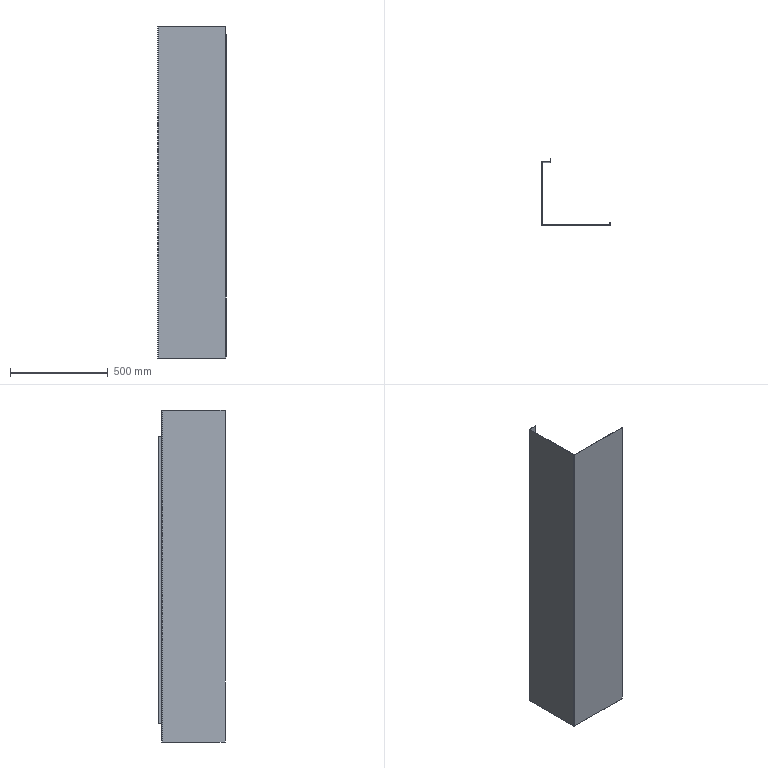Component | SolidWorks | SidePanel-1 | 1 solid | 41 faces | box 350 x 342.5 x 1700 mm | volume 1886748 mm3 | plane 33 | cylinder 8 | commonest cylinder face diameters 1 x4 4 x4
STEP:
#1=COLOUR_RGB('',0.7922,0.8196,0.9333);
#2=FILL_AREA_STYLE_COLOUR('',#1);
#3=FILL_AREA_STYLE('',(#2));
#4=SURFACE_STYLE_FILL_AREA(#3);
#5=SURFACE_SIDE_STYLE('',(#4));
#6=SURFACE_STYLE_USAGE(.BOTH.,#5);
#7=PRESENTATION_STYLE_ASSIGNMENT((#6));
#8=CARTESIAN_POINT('',(7.992,-6.09,65.157));
#9=VERTEX_POINT('',#8);
#10=CARTESIAN_POINT('',(7.992,-6.484,65.157));
#11=VERTEX_POINT('',#10);
#12=CARTESIAN_POINT('',(7.992,-6.563,65.157));
#13=DIRECTION('',(-0.,-1.,0.));
#14=VECTOR('',#13,39.37);
#15=LINE('',#12,#14);
#16=EDGE_CURVE('',#9,#11,#15,.T.);
#17=ORIENTED_EDGE('',*,*,#16,.T.);
#18=CARTESIAN_POINT('',(7.992,-6.484,0.3937));
#19=VERTEX_POINT('',#18);
#20=CARTESIAN_POINT('',(7.992,-6.484,66.929));
#21=DIRECTION('',(0.,0.,-1.));
#22=VECTOR('',#21,39.37);
#23=LINE('',#20,#22);
#24=EDGE_CURVE('',#11,#19,#23,.T.);
#25=ORIENTED_EDGE('',*,*,#24,.T.);
#26=CARTESIAN_POINT('',(7.992,-6.09,0.3937));
#27=VERTEX_POINT('',#26);
#28=CARTESIAN_POINT('',(7.992,-6.563,0.3937));
#29=DIRECTION('',(0.,1.,0.));
#30=VECTOR('',#29,39.37);
#31=LINE('',#28,#30);
#32=EDGE_CURVE('',#19,#27,#31,.T.);
#33=ORIENTED_EDGE('',*,*,#32,.T.);
#34=CARTESIAN_POINT('',(7.992,-6.09,66.929));
#35=DIRECTION('',(0.,0.,-1.));
#36=VECTOR('',#35,39.37);
#37=LINE('',#34,#36);
#38=EDGE_CURVE('',#9,#27,#37,.T.);
#39=ORIENTED_EDGE('',*,*,#38,.F.);
#40=EDGE_LOOP('',(#17,#25,#33,#39));
#41=FACE_OUTER_BOUND('',#40,.T.);
#42=CARTESIAN_POINT('',(7.992,-6.563,66.929));
#43=DIRECTION('',(-1.,0.,0.));
#44=DIRECTION('',(-0.,-1.,0.));
#45=AXIS2_PLACEMENT_3D('',#42,#43,#44);
#46=PLANE('',#45);
#47=ADVANCED_FACE('',(#41),#46,.F.);
#48=CARTESIAN_POINT('',(7.933,-6.09,65.157));
#49=VERTEX_POINT('',#48);
#50=CARTESIAN_POINT('',(7.933,-6.09,0.3937));
#51=VERTEX_POINT('',#50);
#52=CARTESIAN_POINT('',(7.933,-6.09,66.929));
#53=DIRECTION('',(0.,0.,-1.));
#54=VECTOR('',#53,39.37);
#55=LINE('',#52,#54);
#56=EDGE_CURVE('',#49,#51,#55,.T.);
#57=ORIENTED_EDGE('',*,*,#56,.F.);
#58=CARTESIAN_POINT('',(7.933,-6.09,65.157));
#59=DIRECTION('',(1.,-0.,0.));
#60=VECTOR('',#59,39.37);
#61=LINE('',#58,#60);
#62=EDGE_CURVE('',#49,#9,#61,.T.);
#63=ORIENTED_EDGE('',*,*,#62,.T.);
#64=ORIENTED_EDGE('',*,*,#38,.T.);
#65=CARTESIAN_POINT('',(7.933,-6.09,0.3937));
#66=DIRECTION('',(1.,-0.,0.));
#67=VECTOR('',#66,39.37);
#68=LINE('',#65,#67);
#69=EDGE_CURVE('',#51,#27,#68,.T.);
#70=ORIENTED_EDGE('',*,*,#69,.F.);
#71=EDGE_LOOP('',(#57,#63,#64,#70));
#72=FACE_OUTER_BOUND('',#71,.T.);
#73=CARTESIAN_POINT('',(7.933,-6.09,66.929));
#74=DIRECTION('',(0.,1.,0.));
#75=DIRECTION('',(0.,0.,1.));
#76=AXIS2_PLACEMENT_3D('',#73,#74,#75);
#77=PLANE('',#76);
#78=ADVANCED_FACE('',(#72),#77,.T.);
#79=CARTESIAN_POINT('',(7.933,-6.484,65.157));
#80=VERTEX_POINT('',#79);
#81=CARTESIAN_POINT('',(7.933,-6.484,0.3937));
#82=VERTEX_POINT('',#81);
#83=CARTESIAN_POINT('',(7.933,-6.484,66.929));
#84=DIRECTION('',(0.,0.,-1.));
#85=VECTOR('',#84,39.37);
#86=LINE('',#83,#85);
#87=EDGE_CURVE('',#80,#82,#86,.T.);
#88=ORIENTED_EDGE('',*,*,#87,.F.);
#89=CARTESIAN_POINT('',(7.933,-6.563,65.157));
#90=DIRECTION('',(-0.,-1.,0.));
#91=VECTOR('',#90,39.37);
#92=LINE('',#89,#91);
#93=EDGE_CURVE('',#49,#80,#92,.T.);
#94=ORIENTED_EDGE('',*,*,#93,.F.);
#95=ORIENTED_EDGE('',*,*,#56,.T.);
#96=CARTESIAN_POINT('',(7.933,-6.563,0.3937));
#97=DIRECTION('',(0.,1.,0.));
#98=VECTOR('',#97,39.37);
#99=LINE('',#96,#98);
#100=EDGE_CURVE('',#82,#51,#99,.T.);
#101=ORIENTED_EDGE('',*,*,#100,.F.);
#102=EDGE_LOOP('',(#88,#94,#95,#101));
#103=FACE_OUTER_BOUND('',#102,.T.);
#104=CARTESIAN_POINT('',(7.933,-6.563,66.929));
#105=DIRECTION('',(-1.,0.,0.));
#106=DIRECTION('',(-0.,-1.,0.));
#107=AXIS2_PLACEMENT_3D('',#104,#105,#106);
#108=PLANE('',#107);
#109=ADVANCED_FACE('',(#103),#108,.T.);
#110=CARTESIAN_POINT('',(7.913,-6.504,65.157));
#111=VERTEX_POINT('',#110);
#112=CARTESIAN_POINT('',(7.913,-6.504,0.3937));
#113=VERTEX_POINT('',#112);
#114=CARTESIAN_POINT('',(7.913,-6.504,66.929));
#115=DIRECTION('',(0.,0.,-1.));
#116=VECTOR('',#115,39.37);
#117=LINE('',#114,#116);
#118=EDGE_CURVE('',#111,#113,#117,.T.);
#119=ORIENTED_EDGE('',*,*,#118,.F.);
#120=CARTESIAN_POINT('',(7.913,-6.484,65.157));
#121=DIRECTION('',(0.,0.,-1.));
#122=DIRECTION('',(-1.,0.,0.));
#123=AXIS2_PLACEMENT_3D('',#120,#121,#122);
#124=CIRCLE('',#123,0.01969);
#125=EDGE_CURVE('',#80,#111,#124,.T.);
#126=ORIENTED_EDGE('',*,*,#125,.F.);
#127=ORIENTED_EDGE('',*,*,#87,.T.);
#128=CARTESIAN_POINT('',(7.913,-6.484,0.3937));
#129=DIRECTION('',(0.,0.,1.));
#130=DIRECTION('',(-1.,0.,0.));
#131=AXIS2_PLACEMENT_3D('',#128,#129,#130);
#132=CIRCLE('',#131,0.01969);
#133=EDGE_CURVE('',#113,#82,#132,.T.);
#134=ORIENTED_EDGE('',*,*,#133,.F.);
#135=EDGE_LOOP('',(#119,#126,#127,#134));
#136=FACE_OUTER_BOUND('',#135,.T.);
#137=CARTESIAN_POINT('',(7.913,-6.484,66.929));
#138=DIRECTION('',(0.,0.,-1.));
#139=DIRECTION('',(-1.,0.,0.));
#140=AXIS2_PLACEMENT_3D('',#137,#138,#139);
#141=CYLINDRICAL_SURFACE('',#140,0.01969);
#142=ADVANCED_FACE('',(#136),#141,.F.);
#143=CARTESIAN_POINT('',(7.913,-6.563,65.157));
#144=VERTEX_POINT('',#143);
#145=CARTESIAN_POINT('',(7.913,-6.484,65.157));
#146=DIRECTION('',(0.,0.,-1.));
#147=DIRECTION('',(-1.,0.,0.));
#148=AXIS2_PLACEMENT_3D('',#145,#146,#147);
#149=CIRCLE('',#148,0.07874);
#150=EDGE_CURVE('',#11,#144,#149,.T.);
#151=ORIENTED_EDGE('',*,*,#150,.T.);
#152=CARTESIAN_POINT('',(7.913,-6.563,0.3937));
#153=VERTEX_POINT('',#152);
#154=CARTESIAN_POINT('',(7.913,-6.563,66.929));
#155=DIRECTION('',(0.,0.,-1.));
#156=VECTOR('',#155,39.37);
#157=LINE('',#154,#156);
#158=EDGE_CURVE('',#144,#153,#157,.T.);
#159=ORIENTED_EDGE('',*,*,#158,.T.);
#160=CARTESIAN_POINT('',(7.913,-6.484,0.3937));
#161=DIRECTION('',(0.,0.,1.));
#162=DIRECTION('',(1.,0.,0.));
#163=AXIS2_PLACEMENT_3D('',#160,#161,#162);
#164=CIRCLE('',#163,0.07874);
#165=EDGE_CURVE('',#153,#19,#164,.T.);
#166=ORIENTED_EDGE('',*,*,#165,.T.);
#167=ORIENTED_EDGE('',*,*,#24,.F.);
#168=EDGE_LOOP('',(#151,#159,#166,#167));
#169=FACE_OUTER_BOUND('',#168,.T.);
#170=CARTESIAN_POINT('',(7.913,-6.484,66.929));
#171=DIRECTION('',(0.,0.,-1.));
#172=DIRECTION('',(-1.,0.,0.));
#173=AXIS2_PLACEMENT_3D('',#170,#171,#172);
#174=CYLINDRICAL_SURFACE('',#173,0.07874);
#175=ADVANCED_FACE('',(#169),#174,.T.);
#176=CARTESIAN_POINT('',(-4.016,6.252,3.74));
#177=VERTEX_POINT('',#176);
#178=CARTESIAN_POINT('',(-4.016,6.922,3.74));
#179=VERTEX_POINT('',#178);
#180=CARTESIAN_POINT('',(-4.016,6.174,3.74));
#181=DIRECTION('',(0.,1.,0.));
#182=VECTOR('',#181,39.37);
#183=LINE('',#180,#182);
#184=EDGE_CURVE('',#177,#179,#183,.T.);
#185=ORIENTED_EDGE('',*,*,#184,.F.);
#186=CARTESIAN_POINT('',(-4.075,6.252,3.74));
#187=VERTEX_POINT('',#186);
#188=CARTESIAN_POINT('',(-4.016,6.252,3.74));
#189=DIRECTION('',(-1.,0.,-0.));
#190=VECTOR('',#189,39.37);
#191=LINE('',#188,#190);
#192=EDGE_CURVE('',#177,#187,#191,.T.);
#193=ORIENTED_EDGE('',*,*,#192,.T.);
#194=CARTESIAN_POINT('',(-4.075,6.922,3.74));
#195=VERTEX_POINT('',#194);
#196=CARTESIAN_POINT('',(-4.075,6.922,3.74));
#197=DIRECTION('',(0.,-1.,0.));
#198=VECTOR('',#197,39.37);
#199=LINE('',#196,#198);
#200=EDGE_CURVE('',#195,#187,#199,.T.);
#201=ORIENTED_EDGE('',*,*,#200,.F.);
#202=CARTESIAN_POINT('',(-4.095,6.922,3.74));
#203=DIRECTION('',(1.,0.,0.));
#204=VECTOR('',#203,39.37);
#205=LINE('',#202,#204);
#206=EDGE_CURVE('',#195,#179,#205,.T.);
#207=ORIENTED_EDGE('',*,*,#206,.T.);
#208=EDGE_LOOP('',(#185,#193,#201,#207));
#209=FACE_OUTER_BOUND('',#208,.T.);
#210=CARTESIAN_POINT('',(-4.095,6.174,3.74));
#211=DIRECTION('',(0.,0.,1.));
#212=DIRECTION('',(1.,0.,0.));
#213=AXIS2_PLACEMENT_3D('',#210,#211,#212);
#214=PLANE('',#213);
#215=ADVANCED_FACE('',(#209),#214,.F.);
#216=CARTESIAN_POINT('',(-4.095,6.233,0.));
#217=VERTEX_POINT('',#216);
#218=CARTESIAN_POINT('',(-5.709,6.233,0.));
#219=VERTEX_POINT('',#218);
#220=CARTESIAN_POINT('',(-4.075,6.233,0.));
#221=DIRECTION('',(-1.,0.,0.));
#222=VECTOR('',#221,39.37);
#223=LINE('',#220,#222);
#224=EDGE_CURVE('',#217,#219,#223,.T.);
#225=ORIENTED_EDGE('',*,*,#224,.F.);
#226=CARTESIAN_POINT('',(-4.095,6.174,0.));
#227=VERTEX_POINT('',#226);
#228=CARTESIAN_POINT('',(-4.095,6.233,0.));
#229=DIRECTION('',(0.,-1.,0.));
#230=VECTOR('',#229,39.37);
#231=LINE('',#228,#230);
#232=EDGE_CURVE('',#217,#227,#231,.T.);
#233=ORIENTED_EDGE('',*,*,#232,.T.);
#234=CARTESIAN_POINT('',(-5.709,6.174,0.));
#235=VERTEX_POINT('',#234);
#236=CARTESIAN_POINT('',(-4.075,6.174,0.));
#237=DIRECTION('',(-1.,0.,0.));
#238=VECTOR('',#237,39.37);
#239=LINE('',#236,#238);
#240=EDGE_CURVE('',#227,#235,#239,.T.);
#241=ORIENTED_EDGE('',*,*,#240,.T.);
#242=CARTESIAN_POINT('',(-5.709,6.174,0.));
#243=DIRECTION('',(0.,1.,0.));
#244=VECTOR('',#243,39.37);
#245=LINE('',#242,#244);
#246=EDGE_CURVE('',#235,#219,#245,.T.);
#247=ORIENTED_EDGE('',*,*,#246,.T.);
#248=EDGE_LOOP('',(#225,#233,#241,#247));
#249=FACE_OUTER_BOUND('',#248,.T.);
#250=CARTESIAN_POINT('',(-4.016,6.252,0.));
#251=DIRECTION('',(0.,0.,-1.));
#252=DIRECTION('',(-1.,0.,0.));
#253=AXIS2_PLACEMENT_3D('',#250,#251,#252);
#254=PLANE('',#253);
#255=ADVANCED_FACE('',(#249),#254,.T.);
#256=CARTESIAN_POINT('',(-5.709,6.233,66.929));
#257=VERTEX_POINT('',#256);
#258=CARTESIAN_POINT('',(-5.709,6.174,66.929));
#259=VERTEX_POINT('',#258);
#260=CARTESIAN_POINT('',(-5.709,6.233,66.929));
#261=DIRECTION('',(0.,-1.,0.));
#262=VECTOR('',#261,39.37);
#263=LINE('',#260,#262);
#264=EDGE_CURVE('',#257,#259,#263,.T.);
#265=ORIENTED_EDGE('',*,*,#264,.F.);
#266=CARTESIAN_POINT('',(-5.788,6.154,66.929));
#267=VERTEX_POINT('',#266);
#268=CARTESIAN_POINT('',(-5.709,6.154,66.929));
#269=DIRECTION('',(0.,0.,1.));
#270=DIRECTION('',(-1.,0.,0.));
#271=AXIS2_PLACEMENT_3D('',#268,#269,#270);
#272=CIRCLE('',#271,0.07874);
#273=EDGE_CURVE('',#257,#267,#272,.T.);
#274=ORIENTED_EDGE('',*,*,#273,.T.);
#275=CARTESIAN_POINT('',(-5.729,6.154,66.929));
#276=VERTEX_POINT('',#275);
#277=CARTESIAN_POINT('',(-5.729,6.154,66.929));
#278=DIRECTION('',(-1.,0.,0.));
#279=VECTOR('',#278,39.37);
#280=LINE('',#277,#279);
#281=EDGE_CURVE('',#276,#267,#280,.T.);
#282=ORIENTED_EDGE('',*,*,#281,.F.);
#283=CARTESIAN_POINT('',(-5.709,6.154,66.929));
#284=DIRECTION('',(0.,0.,1.));
#285=DIRECTION('',(1.,0.,0.));
#286=AXIS2_PLACEMENT_3D('',#283,#284,#285);
#287=CIRCLE('',#286,0.01969);
#288=EDGE_CURVE('',#259,#276,#287,.T.);
#289=ORIENTED_EDGE('',*,*,#288,.F.);
#290=EDGE_LOOP('',(#265,#274,#282,#289));
#291=FACE_OUTER_BOUND('',#290,.T.);
#292=CARTESIAN_POINT('',(-5.709,6.233,66.929));
#293=DIRECTION('',(0.,0.,1.));
#294=DIRECTION('',(1.,0.,0.));
#295=AXIS2_PLACEMENT_3D('',#292,#293,#294);
#296=PLANE('',#295);
#297=ADVANCED_FACE('',(#291),#296,.T.);
#298=CARTESIAN_POINT('',(-4.095,6.233,66.929));
#299=VERTEX_POINT('',#298);
#300=CARTESIAN_POINT('',(-4.075,6.233,66.929));
#301=DIRECTION('',(-1.,0.,0.));
#302=VECTOR('',#301,39.37);
#303=LINE('',#300,#302);
#304=EDGE_CURVE('',#299,#257,#303,.T.);
#305=ORIENTED_EDGE('',*,*,#304,.T.);
#306=ORIENTED_EDGE('',*,*,#264,.T.);
#307=CARTESIAN_POINT('',(-4.095,6.174,66.929));
#308=VERTEX_POINT('',#307);
#309=CARTESIAN_POINT('',(-4.075,6.174,66.929));
#310=DIRECTION('',(-1.,0.,0.));
#311=VECTOR('',#310,39.37);
#312=LINE('',#309,#311);
#313=EDGE_CURVE('',#308,#259,#312,.T.);
#314=ORIENTED_EDGE('',*,*,#313,.F.);
#315=CARTESIAN_POINT('',(-4.095,6.174,66.929));
#316=DIRECTION('',(0.,1.,0.));
#317=VECTOR('',#316,39.37);
#318=LINE('',#315,#317);
#319=EDGE_CURVE('',#308,#299,#318,.T.);
#320=ORIENTED_EDGE('',*,*,#319,.T.);
#321=EDGE_LOOP('',(#305,#306,#314,#320));
#322=FACE_OUTER_BOUND('',#321,.T.);
#323=CARTESIAN_POINT('',(-5.729,6.154,66.929));
#324=DIRECTION('',(0.,0.,1.));
#325=DIRECTION('',(1.,0.,0.));
#326=AXIS2_PLACEMENT_3D('',#323,#324,#325);
#327=PLANE('',#326);
#328=ADVANCED_FACE('',(#322),#327,.T.);
#329=CARTESIAN_POINT('',(-5.788,6.154,0.));
#330=VERTEX_POINT('',#329);
#331=CARTESIAN_POINT('',(-5.729,6.154,0.));
#332=VERTEX_POINT('',#331);
#333=CARTESIAN_POINT('',(-5.788,6.154,0.));
#334=DIRECTION('',(1.,0.,0.));
#335=VECTOR('',#334,39.37);
#336=LINE('',#333,#335);
#337=EDGE_CURVE('',#330,#332,#336,.T.);
#338=ORIENTED_EDGE('',*,*,#337,.F.);
#339=CARTESIAN_POINT('',(-5.709,6.154,0.));
#340=DIRECTION('',(0.,0.,1.));
#341=DIRECTION('',(-1.,0.,0.));
#342=AXIS2_PLACEMENT_3D('',#339,#340,#341);
#343=CIRCLE('',#342,0.07874);
#344=EDGE_CURVE('',#219,#330,#343,.T.);
#345=ORIENTED_EDGE('',*,*,#344,.F.);
#346=ORIENTED_EDGE('',*,*,#246,.F.);
#347=CARTESIAN_POINT('',(-5.709,6.154,0.));
#348=DIRECTION('',(0.,0.,1.));
#349=DIRECTION('',(1.,0.,0.));
#350=AXIS2_PLACEMENT_3D('',#347,#348,#349);
#351=CIRCLE('',#350,0.01969);
#352=EDGE_CURVE('',#235,#332,#351,.T.);
#353=ORIENTED_EDGE('',*,*,#352,.T.);
#354=EDGE_LOOP('',(#338,#345,#346,#353));
#355=FACE_OUTER_BOUND('',#354,.T.);
#356=CARTESIAN_POINT('',(-5.788,6.154,0.));
#357=DIRECTION('',(0.,0.,-1.));
#358=DIRECTION('',(-1.,0.,0.));
#359=AXIS2_PLACEMENT_3D('',#356,#357,#358);
#360=PLANE('',#359);
#361=ADVANCED_FACE('',(#355),#360,.T.);
#362=CARTESIAN_POINT('',(-5.788,-6.484,0.));
#363=VERTEX_POINT('',#362);
#364=CARTESIAN_POINT('',(-5.788,6.233,0.));
#365=DIRECTION('',(0.,-1.,0.));
#366=VECTOR('',#365,39.37);
#367=LINE('',#364,#366);
#368=EDGE_CURVE('',#330,#363,#367,.T.);
#369=ORIENTED_EDGE('',*,*,#368,.F.);
#370=ORIENTED_EDGE('',*,*,#337,.T.);
#371=CARTESIAN_POINT('',(-5.729,-6.484,0.));
#372=VERTEX_POINT('',#371);
#373=CARTESIAN_POINT('',(-5.729,6.233,0.));
#374=DIRECTION('',(0.,-1.,0.));
#375=VECTOR('',#374,39.37);
#376=LINE('',#373,#375);
#377=EDGE_CURVE('',#332,#372,#376,.T.);
#378=ORIENTED_EDGE('',*,*,#377,.T.);
#379=CARTESIAN_POINT('',(-5.729,-6.484,0.));
#380=DIRECTION('',(-1.,0.,0.));
#381=VECTOR('',#380,39.37);
#382=LINE('',#379,#381);
#383=EDGE_CURVE('',#372,#363,#382,.T.);
#384=ORIENTED_EDGE('',*,*,#383,.T.);
#385=EDGE_LOOP('',(#369,#370,#378,#384));
#386=FACE_OUTER_BOUND('',#385,.T.);
#387=CARTESIAN_POINT('',(-5.709,6.174,0.));
#388=DIRECTION('',(0.,0.,-1.));
#389=DIRECTION('',(-1.,0.,0.));
#390=AXIS2_PLACEMENT_3D('',#387,#388,#389);
#391=PLANE('',#390);
#392=ADVANCED_FACE('',(#386),#391,.T.);
#393=CARTESIAN_POINT('',(-5.788,-6.484,66.929));
#394=VERTEX_POINT('',#393);
#395=CARTESIAN_POINT('',(-5.729,-6.484,66.929));
#396=VERTEX_POINT('',#395);
#397=CARTESIAN_POINT('',(-5.788,-6.484,66.929));
#398=DIRECTION('',(1.,0.,0.));
#399=VECTOR('',#398,39.37);
#400=LINE('',#397,#399);
#401=EDGE_CURVE('',#394,#396,#400,.T.);
#402=ORIENTED_EDGE('',*,*,#401,.F.);
#403=CARTESIAN_POINT('',(-5.709,-6.563,66.929));
#404=VERTEX_POINT('',#403);
#405=CARTESIAN_POINT('',(-5.709,-6.484,66.929));
#406=DIRECTION('',(0.,0.,1.));
#407=DIRECTION('',(-1.,0.,0.));
#408=AXIS2_PLACEMENT_3D('',#405,#406,#407);
#409=CIRCLE('',#408,0.07874);
#410=EDGE_CURVE('',#394,#404,#409,.T.);
#411=ORIENTED_EDGE('',*,*,#410,.T.);
#412=CARTESIAN_POINT('',(-5.709,-6.504,66.929));
#413=VERTEX_POINT('',#412);
#414=CARTESIAN_POINT('',(-5.709,-6.504,66.929));
#415=DIRECTION('',(0.,-1.,0.));
#416=VECTOR('',#415,39.37);
#417=LINE('',#414,#416);
#418=EDGE_CURVE('',#413,#404,#417,.T.);
#419=ORIENTED_EDGE('',*,*,#418,.F.);
#420=CARTESIAN_POINT('',(-5.709,-6.484,66.929));
#421=DIRECTION('',(0.,0.,1.));
#422=DIRECTION('',(1.,0.,0.));
#423=AXIS2_PLACEMENT_3D('',#420,#421,#422);
#424=CIRCLE('',#423,0.01969);
#425=EDGE_CURVE('',#396,#413,#424,.T.);
#426=ORIENTED_EDGE('',*,*,#425,.F.);
#427=EDGE_LOOP('',(#402,#411,#419,#426));
#428=FACE_OUTER_BOUND('',#427,.T.);
#429=CARTESIAN_POINT('',(-5.788,-6.484,66.929));
#430=DIRECTION('',(0.,0.,1.));
#431=DIRECTION('',(1.,0.,0.));
#432=AXIS2_PLACEMENT_3D('',#429,#430,#431);
#433=PLANE('',#432);
#434=ADVANCED_FACE('',(#428),#433,.T.);
#435=CARTESIAN_POINT('',(-5.788,6.233,66.929));
#436=DIRECTION('',(0.,-1.,0.));
#437=VECTOR('',#436,39.37);
#438=LINE('',#435,#437);
#439=EDGE_CURVE('',#267,#394,#438,.T.);
#440=ORIENTED_EDGE('',*,*,#439,.T.);
#441=ORIENTED_EDGE('',*,*,#401,.T.);
#442=CARTESIAN_POINT('',(-5.729,6.233,66.929));
#443=DIRECTION('',(0.,-1.,0.));
#444=VECTOR('',#443,39.37);
#445=LINE('',#442,#444);
#446=EDGE_CURVE('',#276,#396,#445,.T.);
#447=ORIENTED_EDGE('',*,*,#446,.F.);
#448=ORIENTED_EDGE('',*,*,#281,.T.);
#449=EDGE_LOOP('',(#440,#441,#447,#448));
#450=FACE_OUTER_BOUND('',#449,.T.);
#451=CARTESIAN_POINT('',(-5.709,-6.504,66.929));
#452=DIRECTION('',(0.,0.,1.));
#453=DIRECTION('',(1.,0.,0.));
#454=AXIS2_PLACEMENT_3D('',#451,#452,#453);
#455=PLANE('',#454);
#456=ADVANCED_FACE('',(#450),#455,.T.);
#457=CARTESIAN_POINT('',(-5.709,-6.563,0.));
#458=VERTEX_POINT('',#457);
#459=CARTESIAN_POINT('',(-5.709,-6.504,0.));
#460=VERTEX_POINT('',#459);
#461=CARTESIAN_POINT('',(-5.709,-6.563,0.));
#462=DIRECTION('',(0.,1.,0.));
#463=VECTOR('',#462,39.37);
#464=LINE('',#461,#463);
#465=EDGE_CURVE('',#458,#460,#464,.T.);
#466=ORIENTED_EDGE('',*,*,#465,.F.);
#467=CARTESIAN_POINT('',(-5.709,-6.484,0.));
#468=DIRECTION('',(0.,0.,1.));
#469=DIRECTION('',(-1.,0.,0.));
#470=AXIS2_PLACEMENT_3D('',#467,#468,#469);
#471=CIRCLE('',#470,0.07874);
#472=EDGE_CURVE('',#363,#458,#471,.T.);
#473=ORIENTED_EDGE('',*,*,#472,.F.);
#474=ORIENTED_EDGE('',*,*,#383,.F.);
#475=CARTESIAN_POINT('',(-5.709,-6.484,0.));
#476=DIRECTION('',(0.,0.,1.));
#477=DIRECTION('',(1.,0.,0.));
#478=AXIS2_PLACEMENT_3D('',#475,#476,#477);
#479=CIRCLE('',#478,0.01969);
#480=EDGE_CURVE('',#372,#460,#479,.T.);
#481=ORIENTED_EDGE('',*,*,#480,.T.);
#482=EDGE_LOOP('',(#466,#473,#474,#481));
#483=FACE_OUTER_BOUND('',#482,.T.);
#484=CARTESIAN_POINT('',(-5.709,-6.563,0.));
#485=DIRECTION('',(0.,0.,-1.));
#486=DIRECTION('',(-1.,0.,0.));
#487=AXIS2_PLACEMENT_3D('',#484,#485,#486);
#488=PLANE('',#487);
#489=ADVANCED_FACE('',(#483),#488,.T.);
#490=CARTESIAN_POINT('',(7.913,-6.563,0.));
#491=VERTEX_POINT('',#490);
#492=CARTESIAN_POINT('',(-5.788,-6.563,0.));
#493=DIRECTION('',(1.,0.,0.));
#494=VECTOR('',#493,39.37);
#495=LINE('',#492,#494);
#496=EDGE_CURVE('',#458,#491,#495,.T.);
#497=ORIENTED_EDGE('',*,*,#496,.F.);
#498=ORIENTED_EDGE('',*,*,#465,.T.);
#499=CARTESIAN_POINT('',(7.913,-6.504,0.));
#500=VERTEX_POINT('',#499);
#501=CARTESIAN_POINT('',(-5.788,-6.504,0.));
#502=DIRECTION('',(1.,0.,0.));
#503=VECTOR('',#502,39.37);
#504=LINE('',#501,#503);
#505=EDGE_CURVE('',#460,#500,#504,.T.);
#506=ORIENTED_EDGE('',*,*,#505,.T.);
#507=CARTESIAN_POINT('',(7.913,-6.504,0.));
#508=DIRECTION('',(0.,-1.,0.));
#509=VECTOR('',#508,39.37);
#510=LINE('',#507,#509);
#511=EDGE_CURVE('',#500,#491,#510,.T.);
#512=ORIENTED_EDGE('',*,*,#511,.T.);
#513=EDGE_LOOP('',(#497,#498,#506,#512));
#514=FACE_OUTER_BOUND('',#513,.T.);
#515=CARTESIAN_POINT('',(-5.729,-6.484,0.));
#516=DIRECTION('',(0.,0.,-1.));
#517=DIRECTION('',(-1.,0.,0.));
#518=AXIS2_PLACEMENT_3D('',#515,#516,#517);
#519=PLANE('',#518);
#520=ADVANCED_FACE('',(#514),#519,.T.);
#521=CARTESIAN_POINT('',(7.913,-6.563,66.929));
#522=VERTEX_POINT('',#521);
#523=CARTESIAN_POINT('',(-5.788,-6.563,66.929));
#524=DIRECTION('',(1.,0.,0.));
#525=VECTOR('',#524,39.37);
#526=LINE('',#523,#525);
#527=EDGE_CURVE('',#404,#522,#526,.T.);
#528=ORIENTED_EDGE('',*,*,#527,.T.);
#529=CARTESIAN_POINT('',(7.913,-6.504,66.929));
#530=VERTEX_POINT('',#529);
#531=CARTESIAN_POINT('',(7.913,-6.563,66.929));
#532=DIRECTION('',(0.,1.,0.));
#533=VECTOR('',#532,39.37);
#534=LINE('',#531,#533);
#535=EDGE_CURVE('',#522,#530,#534,.T.);
#536=ORIENTED_EDGE('',*,*,#535,.T.);
#537=CARTESIAN_POINT('',(-5.788,-6.504,66.929));
#538=DIRECTION('',(1.,0.,0.));
#539=VECTOR('',#538,39.37);
#540=LINE('',#537,#539);
#541=EDGE_CURVE('',#413,#530,#540,.T.);
#542=ORIENTED_EDGE('',*,*,#541,.F.);
#543=ORIENTED_EDGE('',*,*,#418,.T.);
#544=EDGE_LOOP('',(#528,#536,#542,#543));
#545=FACE_OUTER_BOUND('',#544,.T.);
#546=CARTESIAN_POINT('',(7.933,-6.484,66.929));
#547=DIRECTION('',(0.,0.,1.));
#548=DIRECTION('',(1.,0.,0.));
#549=AXIS2_PLACEMENT_3D('',#546,#547,#548);
#550=PLANE('',#549);
#551=ADVANCED_FACE('',(#545),#550,.T.);
#552=ORIENTED_EDGE('',*,*,#505,.F.);
#553=CARTESIAN_POINT('',(-5.709,-6.504,66.929));
#554=DIRECTION('',(0.,0.,-1.));
#555=VECTOR('',#554,39.37);
#556=LINE('',#553,#555);
#557=EDGE_CURVE('',#413,#460,#556,.T.);
#558=ORIENTED_EDGE('',*,*,#557,.F.);
#559=ORIENTED_EDGE('',*,*,#541,.T.);
#560=CARTESIAN_POINT('',(7.913,-6.504,66.929));
#561=DIRECTION('',(0.,0.,-1.));
#562=VECTOR('',#561,39.37);
#563=LINE('',#560,#562);
#564=EDGE_CURVE('',#530,#111,#563,.T.);
#565=ORIENTED_EDGE('',*,*,#564,.T.);
#566=ORIENTED_EDGE('',*,*,#118,.T.);
#567=CARTESIAN_POINT('',(7.913,-6.504,0.));
#568=DIRECTION('',(0.,0.,-1.));
#569=VECTOR('',#568,39.37);
#570=LINE('',#567,#569);
#571=EDGE_CURVE('',#113,#500,#570,.T.);
#572=ORIENTED_EDGE('',*,*,#571,.T.);
#573=EDGE_LOOP('',(#552,#558,#559,#565,#566,#572));
#574=FACE_OUTER_BOUND('',#573,.T.);
#575=CARTESIAN_POINT('',(-5.788,-6.504,66.929));
#576=DIRECTION('',(0.,1.,0.));
#577=DIRECTION('',(0.,0.,1.));
#578=AXIS2_PLACEMENT_3D('',#575,#576,#577);
#579=PLANE('',#578);
#580=ADVANCED_FACE('',(#574),#579,.T.);
#581=ORIENTED_EDGE('',*,*,#480,.F.);
#582=CARTESIAN_POINT('',(-5.729,-6.484,66.929));
#583=DIRECTION('',(0.,0.,-1.));
#584=VECTOR('',#583,39.37);
#585=LINE('',#582,#584);
#586=EDGE_CURVE('',#396,#372,#585,.T.);
#587=ORIENTED_EDGE('',*,*,#586,.F.);
#588=ORIENTED_EDGE('',*,*,#425,.T.);
#589=ORIENTED_EDGE('',*,*,#557,.T.);
#590=EDGE_LOOP('',(#581,#587,#588,#589));
#591=FACE_OUTER_BOUND('',#590,.T.);
#592=CARTESIAN_POINT('',(-5.709,-6.484,66.929));
#593=DIRECTION('',(0.,0.,-1.));
#594=DIRECTION('',(-1.,0.,0.));
#595=AXIS2_PLACEMENT_3D('',#592,#593,#594);
#596=CYLINDRICAL_SURFACE('',#595,0.01969);
#597=ADVANCED_FACE('',(#591),#596,.F.);
#598=ORIENTED_EDGE('',*,*,#377,.F.);
#599=CARTESIAN_POINT('',(-5.729,6.154,66.929));
#600=DIRECTION('',(0.,0.,-1.));
#601=VECTOR('',#600,39.37);
#602=LINE('',#599,#601);
#603=EDGE_CURVE('',#276,#332,#602,.T.);
#604=ORIENTED_EDGE('',*,*,#603,.F.);
#605=ORIENTED_EDGE('',*,*,#446,.T.);
#606=ORIENTED_EDGE('',*,*,#586,.T.);
#607=EDGE_LOOP('',(#598,#604,#605,#606));
#608=FACE_OUTER_BOUND('',#607,.T.);
#609=CARTESIAN_POINT('',(-5.729,6.233,66.929));
#610=DIRECTION('',(1.,0.,0.));
#611=DIRECTION('',(-0.,1.,0.));
#612=AXIS2_PLACEMENT_3D('',#609,#610,#611);
#613=PLANE('',#612);
#614=ADVANCED_FACE('',(#608),#613,.T.);
#615=ORIENTED_EDGE('',*,*,#352,.F.);
#616=CARTESIAN_POINT('',(-5.709,6.174,66.929));
#617=DIRECTION('',(0.,0.,-1.));
#618=VECTOR('',#617,39.37);
#619=LINE('',#616,#618);
#620=EDGE_CURVE('',#259,#235,#619,.T.);
#621=ORIENTED_EDGE('',*,*,#620,.F.);
#622=ORIENTED_EDGE('',*,*,#288,.T.);
#623=ORIENTED_EDGE('',*,*,#603,.T.);
#624=EDGE_LOOP('',(#615,#621,#622,#623));
#625=FACE_OUTER_BOUND('',#624,.T.);
#626=CARTESIAN_POINT('',(-5.709,6.154,66.929));
#627=DIRECTION('',(0.,0.,-1.));
#628=DIRECTION('',(-1.,0.,0.));
#629=AXIS2_PLACEMENT_3D('',#626,#627,#628);
#630=CYLINDRICAL_SURFACE('',#629,0.01969);
#631=ADVANCED_FACE('',(#625),#630,.F.);
#632=ORIENTED_EDGE('',*,*,#240,.F.);
#633=CARTESIAN_POINT('',(-4.095,6.174,3.74));
#634=VERTEX_POINT('',#633);
#635=CARTESIAN_POINT('',(-4.095,6.174,0.));
#636=DIRECTION('',(0.,0.,1.));
#637=VECTOR('',#636,39.37);
#638=LINE('',#635,#637);
#639=EDGE_CURVE('',#227,#634,#638,.T.);
#640=ORIENTED_EDGE('',*,*,#639,.T.);
#641=CARTESIAN_POINT('',(-4.095,6.174,61.614));
#642=VERTEX_POINT('',#641);
#643=CARTESIAN_POINT('',(-4.095,6.174,66.929));
#644=DIRECTION('',(0.,0.,-1.));
#645=VECTOR('',#644,39.37);
#646=LINE('',#643,#645);
#647=EDGE_CURVE('',#642,#634,#646,.T.);
#648=ORIENTED_EDGE('',*,*,#647,.F.);
#649=CARTESIAN_POINT('',(-4.095,6.174,66.929));
#650=DIRECTION('',(0.,0.,-1.));
#651=VECTOR('',#650,39.37);
#652=LINE('',#649,#651);
#653=EDGE_CURVE('',#308,#642,#652,.T.);
#654=ORIENTED_EDGE('',*,*,#653,.F.);
#655=ORIENTED_EDGE('',*,*,#313,.T.);
#656=ORIENTED_EDGE('',*,*,#620,.T.);
#657=EDGE_LOOP('',(#632,#640,#648,#654,#655,#656));
#658=FACE_OUTER_BOUND('',#657,.T.);
#659=CARTESIAN_POINT('',(-4.075,6.174,66.929));
#660=DIRECTION('',(-0.,-1.,0.));
#661=DIRECTION('',(1.,-0.,0.));
#662=AXIS2_PLACEMENT_3D('',#659,#660,#661);
#663=PLANE('',#662);
#664=ADVANCED_FACE('',(#658),#663,.T.);
#665=CARTESIAN_POINT('',(-4.016,6.252,61.614));
#666=VERTEX_POINT('',#665);
#667=CARTESIAN_POINT('',(-4.095,6.252,61.614));
#668=DIRECTION('',(0.,0.,1.));
#669=DIRECTION('',(-1.,0.,0.));
#670=AXIS2_PLACEMENT_3D('',#667,#668,#669);
#671=CIRCLE('',#670,0.07874);
#672=EDGE_CURVE('',#642,#666,#671,.T.);
#673=ORIENTED_EDGE('',*,*,#672,.F.);
#674=ORIENTED_EDGE('',*,*,#647,.T.);
#675=CARTESIAN_POINT('',(-4.095,6.252,3.74));
#676=DIRECTION('',(0.,0.,-1.));
#677=DIRECTION('',(1.,0.,0.));
#678=AXIS2_PLACEMENT_3D('',#675,#676,#677);
#679=CIRCLE('',#678,0.07874);
#680=EDGE_CURVE('',#177,#634,#679,.T.);
#681=ORIENTED_EDGE('',*,*,#680,.F.);
#682=CARTESIAN_POINT('',(-4.016,6.252,66.929));
#683=DIRECTION('',(0.,0.,-1.));
#684=VECTOR('',#683,39.37);
#685=LINE('',#682,#684);
#686=EDGE_CURVE('',#666,#177,#685,.T.);
#687=ORIENTED_EDGE('',*,*,#686,.F.);
#688=EDGE_LOOP('',(#673,#674,#681,#687));
#689=FACE_OUTER_BOUND('',#688,.T.);
#690=CARTESIAN_POINT('',(-4.095,6.252,66.929));
#691=DIRECTION('',(0.,0.,-1.));
#692=DIRECTION('',(-1.,0.,0.));
#693=AXIS2_PLACEMENT_3D('',#690,#691,#692);
#694=CYLINDRICAL_SURFACE('',#693,0.07874);
#695=ADVANCED_FACE('',(#689),#694,.T.);
#696=CARTESIAN_POINT('',(-4.016,6.922,61.614));
#697=VERTEX_POINT('',#696);
#698=CARTESIAN_POINT('',(-4.016,6.174,61.614));
#699=DIRECTION('',(0.,1.,0.));
#700=VECTOR('',#699,39.37);
#701=LINE('',#698,#700);
#702=EDGE_CURVE('',#666,#697,#701,.T.);
#703=ORIENTED_EDGE('',*,*,#702,.F.);
#704=ORIENTED_EDGE('',*,*,#686,.T.);
#705=ORIENTED_EDGE('',*,*,#184,.T.);
#706=CARTESIAN_POINT('',(-4.016,6.922,66.929));
#707=DIRECTION('',(0.,0.,-1.));
#708=VECTOR('',#707,39.37);
#709=LINE('',#706,#708);
#710=EDGE_CURVE('',#697,#179,#709,.T.);
#711=ORIENTED_EDGE('',*,*,#710,.F.);
#712=EDGE_LOOP('',(#703,#704,#705,#711));
#713=FACE_OUTER_BOUND('',#712,.T.);
#714=CARTESIAN_POINT('',(-4.016,6.922,66.929));
#715=DIRECTION('',(1.,0.,0.));
#716=DIRECTION('',(-0.,1.,0.));
#717=AXIS2_PLACEMENT_3D('',#714,#715,#716);
#718=PLANE('',#717);
#719=ADVANCED_FACE('',(#713),#718,.T.);
#720=CARTESIAN_POINT('',(-4.075,6.922,61.614));
#721=VERTEX_POINT('',#720);
#722=CARTESIAN_POINT('',(-4.016,6.922,61.614));
#723=DIRECTION('',(-1.,0.,0.));
#724=VECTOR('',#723,39.37);
#725=LINE('',#722,#724);
#726=EDGE_CURVE('',#697,#721,#725,.T.);
#727=ORIENTED_EDGE('',*,*,#726,.F.);
#728=ORIENTED_EDGE('',*,*,#710,.T.);
#729=ORIENTED_EDGE('',*,*,#206,.F.);
#730=CARTESIAN_POINT('',(-4.075,6.922,66.929));
#731=DIRECTION('',(0.,0.,-1.));
#732=VECTOR('',#731,39.37);
#733=LINE('',#730,#732);
#734=EDGE_CURVE('',#721,#195,#733,.T.);
#735=ORIENTED_EDGE('',*,*,#734,.F.);
#736=EDGE_LOOP('',(#727,#728,#729,#735));
#737=FACE_OUTER_BOUND('',#736,.T.);
#738=CARTESIAN_POINT('',(-4.075,6.922,66.929));
#739=DIRECTION('',(0.,1.,0.));
#740=DIRECTION('',(0.,0.,1.));
#741=AXIS2_PLACEMENT_3D('',#738,#739,#740);
#742=PLANE('',#741);
#743=ADVANCED_FACE('',(#737),#742,.T.);
#744=CARTESIAN_POINT('',(-4.075,6.252,61.614));
#745=VERTEX_POINT('',#744);
#746=CARTESIAN_POINT('',(-4.075,6.252,66.929));
#747=DIRECTION('',(0.,0.,-1.));
#748=VECTOR('',#747,39.37);
#749=LINE('',#746,#748);
#750=EDGE_CURVE('',#745,#187,#749,.T.);
#751=ORIENTED_EDGE('',*,*,#750,.F.);
#752=CARTESIAN_POINT('',(-4.075,6.922,61.614));
#753=DIRECTION('',(-0.,1.,0.));
#754=VECTOR('',#753,39.37);
#755=LINE('',#752,#754);
#756=EDGE_CURVE('',#745,#721,#755,.T.);
#757=ORIENTED_EDGE('',*,*,#756,.T.);
#758=ORIENTED_EDGE('',*,*,#734,.T.);
#759=ORIENTED_EDGE('',*,*,#200,.T.);
#760=EDGE_LOOP('',(#751,#757,#758,#759));
#761=FACE_OUTER_BOUND('',#760,.T.);
#762=CARTESIAN_POINT('',(-4.075,6.922,66.929));
#763=DIRECTION('',(1.,0.,0.));
#764=DIRECTION('',(-0.,1.,0.));
#765=AXIS2_PLACEMENT_3D('',#762,#763,#764);
#766=PLANE('',#765);
#767=ADVANCED_FACE('',(#761),#766,.F.);
#768=CARTESIAN_POINT('',(-4.095,6.233,61.614));
#769=VERTEX_POINT('',#768);
#770=CARTESIAN_POINT('',(-4.095,6.233,3.74));
#771=VERTEX_POINT('',#770);
#772=CARTESIAN_POINT('',(-4.095,6.233,66.929));
#773=DIRECTION('',(0.,0.,-1.));
#774=VECTOR('',#773,39.37);
#775=LINE('',#772,#774);
#776=EDGE_CURVE('',#769,#771,#775,.T.);
#777=ORIENTED_EDGE('',*,*,#776,.F.);
#778=CARTESIAN_POINT('',(-4.095,6.252,61.614));
#779=DIRECTION('',(0.,0.,1.));
#780=DIRECTION('',(-1.,0.,0.));
#781=AXIS2_PLACEMENT_3D('',#778,#779,#780);
#782=CIRCLE('',#781,0.01969);
#783=EDGE_CURVE('',#769,#745,#782,.T.);
#784=ORIENTED_EDGE('',*,*,#783,.T.);
#785=ORIENTED_EDGE('',*,*,#750,.T.);
#786=CARTESIAN_POINT('',(-4.095,6.252,3.74));
#787=DIRECTION('',(0.,0.,-1.));
#788=DIRECTION('',(1.,0.,0.));
#789=AXIS2_PLACEMENT_3D('',#786,#787,#788);
#790=CIRCLE('',#789,0.01969);
#791=EDGE_CURVE('',#187,#771,#790,.T.);
#792=ORIENTED_EDGE('',*,*,#791,.T.);
#793=EDGE_LOOP('',(#777,#784,#785,#792));
#794=FACE_OUTER_BOUND('',#793,.T.);
#795=CARTESIAN_POINT('',(-4.095,6.252,66.929));
#796=DIRECTION('',(0.,0.,-1.));
#797=DIRECTION('',(-1.,0.,0.));
#798=AXIS2_PLACEMENT_3D('',#795,#796,#797);
#799=CYLINDRICAL_SURFACE('',#798,0.01969);
#800=ADVANCED_FACE('',(#794),#799,.F.);
#801=ORIENTED_EDGE('',*,*,#224,.T.);
#802=CARTESIAN_POINT('',(-5.709,6.233,66.929));
#803=DIRECTION('',(0.,0.,-1.));
#804=VECTOR('',#803,39.37);
#805=LINE('',#802,#804);
#806=EDGE_CURVE('',#257,#219,#805,.T.);
#807=ORIENTED_EDGE('',*,*,#806,.F.);
#808=ORIENTED_EDGE('',*,*,#304,.F.);
#809=CARTESIAN_POINT('',(-4.095,6.233,66.929));
#810=DIRECTION('',(0.,0.,-1.));
#811=VECTOR('',#810,39.37);
#812=LINE('',#809,#811);
#813=EDGE_CURVE('',#299,#769,#812,.T.);
#814=ORIENTED_EDGE('',*,*,#813,.T.);
#815=ORIENTED_EDGE('',*,*,#776,.T.);
#816=CARTESIAN_POINT('',(-4.095,6.233,66.929));
#817=DIRECTION('',(0.,0.,-1.));
#818=VECTOR('',#817,39.37);
#819=LINE('',#816,#818);
#820=EDGE_CURVE('',#771,#217,#819,.T.);
#821=ORIENTED_EDGE('',*,*,#820,.T.);
#822=EDGE_LOOP('',(#801,#807,#808,#814,#815,#821));
#823=FACE_OUTER_BOUND('',#822,.T.);
#824=CARTESIAN_POINT('',(-4.075,6.233,66.929));
#825=DIRECTION('',(-0.,-1.,0.));
#826=DIRECTION('',(1.,-0.,0.));
#827=AXIS2_PLACEMENT_3D('',#824,#825,#826);
#828=PLANE('',#827);
#829=ADVANCED_FACE('',(#823),#828,.F.);
#830=ORIENTED_EDGE('',*,*,#344,.T.);
#831=CARTESIAN_POINT('',(-5.788,6.154,66.929));
#832=DIRECTION('',(0.,0.,-1.));
#833=VECTOR('',#832,39.37);
#834=LINE('',#831,#833);
#835=EDGE_CURVE('',#267,#330,#834,.T.);
#836=ORIENTED_EDGE('',*,*,#835,.F.);
#837=ORIENTED_EDGE('',*,*,#273,.F.);
#838=ORIENTED_EDGE('',*,*,#806,.T.);
#839=EDGE_LOOP('',(#830,#836,#837,#838));
#840=FACE_OUTER_BOUND('',#839,.T.);
#841=CARTESIAN_POINT('',(-5.709,6.154,66.929));
#842=DIRECTION('',(0.,0.,-1.));
#843=DIRECTION('',(-1.,0.,0.));
#844=AXIS2_PLACEMENT_3D('',#841,#842,#843);
#845=CYLINDRICAL_SURFACE('',#844,0.07874);
#846=ADVANCED_FACE('',(#840),#845,.T.);
#847=ORIENTED_EDGE('',*,*,#368,.T.);
#848=CARTESIAN_POINT('',(-5.788,-6.484,66.929));
#849=DIRECTION('',(0.,0.,-1.));
#850=VECTOR('',#849,39.37);
#851=LINE('',#848,#850);
#852=EDGE_CURVE('',#394,#363,#851,.T.);
#853=ORIENTED_EDGE('',*,*,#852,.F.);
#854=ORIENTED_EDGE('',*,*,#439,.F.);
#855=ORIENTED_EDGE('',*,*,#835,.T.);
#856=EDGE_LOOP('',(#847,#853,#854,#855));
#857=FACE_OUTER_BOUND('',#856,.T.);
#858=CARTESIAN_POINT('',(-5.788,6.233,66.929));
#859=DIRECTION('',(1.,0.,0.));
#860=DIRECTION('',(-0.,1.,0.));
#861=AXIS2_PLACEMENT_3D('',#858,#859,#860);
#862=PLANE('',#861);
#863=ADVANCED_FACE('',(#857),#862,.F.);
#864=ORIENTED_EDGE('',*,*,#472,.T.);
#865=CARTESIAN_POINT('',(-5.709,-6.563,66.929));
#866=DIRECTION('',(0.,0.,-1.));
#867=VECTOR('',#866,39.37);
#868=LINE('',#865,#867);
#869=EDGE_CURVE('',#404,#458,#868,.T.);
#870=ORIENTED_EDGE('',*,*,#869,.F.);
#871=ORIENTED_EDGE('',*,*,#410,.F.);
#872=ORIENTED_EDGE('',*,*,#852,.T.);
#873=EDGE_LOOP('',(#864,#870,#871,#872));
#874=FACE_OUTER_BOUND('',#873,.T.);
#875=CARTESIAN_POINT('',(-5.709,-6.484,66.929));
#876=DIRECTION('',(0.,0.,-1.));
#877=DIRECTION('',(-1.,0.,0.));
#878=AXIS2_PLACEMENT_3D('',#875,#876,#877);
#879=CYLINDRICAL_SURFACE('',#878,0.07874);
#880=ADVANCED_FACE('',(#874),#879,.T.);
#881=ORIENTED_EDGE('',*,*,#496,.T.);
#882=CARTESIAN_POINT('',(7.913,-6.563,66.929));
#883=DIRECTION('',(0.,0.,-1.));
#884=VECTOR('',#883,39.37);
#885=LINE('',#882,#884);
#886=EDGE_CURVE('',#153,#491,#885,.T.);
#887=ORIENTED_EDGE('',*,*,#886,.F.);
#888=ORIENTED_EDGE('',*,*,#158,.F.);
#889=CARTESIAN_POINT('',(7.913,-6.563,66.929));
#890=DIRECTION('',(0.,0.,-1.));
#891=VECTOR('',#890,39.37);
#892=LINE('',#889,#891);
#893=EDGE_CURVE('',#522,#144,#892,.T.);
#894=ORIENTED_EDGE('',*,*,#893,.F.);
#895=ORIENTED_EDGE('',*,*,#527,.F.);
#896=ORIENTED_EDGE('',*,*,#869,.T.);
#897=EDGE_LOOP('',(#881,#887,#888,#894,#895,#896));
#898=FACE_OUTER_BOUND('',#897,.T.);
#899=CARTESIAN_POINT('',(-5.788,-6.563,66.929));
#900=DIRECTION('',(0.,1.,0.));
#901=DIRECTION('',(0.,0.,1.));
#902=AXIS2_PLACEMENT_3D('',#899,#900,#901);
#903=PLANE('',#902);
#904=ADVANCED_FACE('',(#898),#903,.F.);
#905=ORIENTED_EDGE('',*,*,#192,.F.);
#906=ORIENTED_EDGE('',*,*,#680,.T.);
#907=CARTESIAN_POINT('',(-4.095,6.174,3.74));
#908=DIRECTION('',(0.,1.,0.));
#909=VECTOR('',#908,39.37);
#910=LINE('',#907,#909);
#911=EDGE_CURVE('',#634,#771,#910,.T.);
#912=ORIENTED_EDGE('',*,*,#911,.T.);
#913=ORIENTED_EDGE('',*,*,#791,.F.);
#914=EDGE_LOOP('',(#905,#906,#912,#913));
#915=FACE_OUTER_BOUND('',#914,.T.);
#916=CARTESIAN_POINT('',(-4.095,6.174,3.74));
#917=DIRECTION('',(0.,0.,1.));
#918=DIRECTION('',(1.,0.,0.));
#919=AXIS2_PLACEMENT_3D('',#916,#917,#918);
#920=PLANE('',#919);
#921=ADVANCED_FACE('',(#915),#920,.F.);
#922=ORIENTED_EDGE('',*,*,#911,.F.);
#923=ORIENTED_EDGE('',*,*,#639,.F.);
#924=ORIENTED_EDGE('',*,*,#232,.F.);
#925=ORIENTED_EDGE('',*,*,#820,.F.);
#926=EDGE_LOOP('',(#922,#923,#924,#925));
#927=FACE_OUTER_BOUND('',#926,.T.);
#928=CARTESIAN_POINT('',(-4.095,6.174,0.));
#929=DIRECTION('',(-1.,0.,0.));
#930=DIRECTION('',(0.,0.,1.));
#931=AXIS2_PLACEMENT_3D('',#928,#929,#930);
#932=PLANE('',#931);
#933=ADVANCED_FACE('',(#927),#932,.F.);
#934=ORIENTED_EDGE('',*,*,#672,.T.);
#935=ORIENTED_EDGE('',*,*,#702,.T.);
#936=ORIENTED_EDGE('',*,*,#726,.T.);
#937=ORIENTED_EDGE('',*,*,#756,.F.);
#938=ORIENTED_EDGE('',*,*,#783,.F.);
#939=CARTESIAN_POINT('',(-4.095,6.174,61.614));
#940=DIRECTION('',(0.,1.,0.));
#941=VECTOR('',#940,39.37);
#942=LINE('',#939,#941);
#943=EDGE_CURVE('',#642,#769,#942,.T.);
#944=ORIENTED_EDGE('',*,*,#943,.F.);
#945=EDGE_LOOP('',(#934,#935,#936,#937,#938,#944));
#946=FACE_OUTER_BOUND('',#945,.T.);
#947=CARTESIAN_POINT('',(-4.016,6.174,61.614));
#948=DIRECTION('',(0.,0.,-1.));
#949=DIRECTION('',(-1.,0.,0.));
#950=AXIS2_PLACEMENT_3D('',#947,#948,#949);
#951=PLANE('',#950);
#952=ADVANCED_FACE('',(#946),#951,.F.);
#953=ORIENTED_EDGE('',*,*,#319,.F.);
#954=ORIENTED_EDGE('',*,*,#653,.T.);
#955=ORIENTED_EDGE('',*,*,#943,.T.);
#956=ORIENTED_EDGE('',*,*,#813,.F.);
#957=EDGE_LOOP('',(#953,#954,#955,#956));
#958=FACE_OUTER_BOUND('',#957,.T.);
#959=CARTESIAN_POINT('',(-4.095,6.174,66.929));
#960=DIRECTION('',(-1.,0.,0.));
#961=DIRECTION('',(0.,0.,1.));
#962=AXIS2_PLACEMENT_3D('',#959,#960,#961);
#963=PLANE('',#962);
#964=ADVANCED_FACE('',(#958),#963,.F.);
#965=ORIENTED_EDGE('',*,*,#100,.T.);
#966=ORIENTED_EDGE('',*,*,#69,.T.);
#967=ORIENTED_EDGE('',*,*,#32,.F.);
#968=CARTESIAN_POINT('',(7.933,-6.484,0.3937));
#969=DIRECTION('',(1.,-0.,0.));
#970=VECTOR('',#969,39.37);
#971=LINE('',#968,#970);
#972=EDGE_CURVE('',#82,#19,#971,.T.);
#973=ORIENTED_EDGE('',*,*,#972,.F.);
#974=EDGE_LOOP('',(#965,#966,#967,#973));
#975=FACE_OUTER_BOUND('',#974,.T.);
#976=CARTESIAN_POINT('',(7.933,-6.563,0.3937));
#977=DIRECTION('',(0.,0.,1.));
#978=DIRECTION('',(0.,1.,0.));
#979=AXIS2_PLACEMENT_3D('',#976,#977,#978);
#980=PLANE('',#979);
#981=ADVANCED_FACE('',(#975),#980,.F.);
#982=ORIENTED_EDGE('',*,*,#972,.T.);
#983=ORIENTED_EDGE('',*,*,#165,.F.);
#984=CARTESIAN_POINT('',(7.913,-6.504,0.3937));
#985=DIRECTION('',(0.,-1.,0.));
#986=VECTOR('',#985,39.37);
#987=LINE('',#984,#986);
#988=EDGE_CURVE('',#113,#153,#987,.T.);
#989=ORIENTED_EDGE('',*,*,#988,.F.);
#990=ORIENTED_EDGE('',*,*,#133,.T.);
#991=EDGE_LOOP('',(#982,#983,#989,#990));
#992=FACE_OUTER_BOUND('',#991,.T.);
#993=CARTESIAN_POINT('',(7.913,-6.484,0.3937));
#994=DIRECTION('',(0.,0.,-1.));
#995=DIRECTION('',(-1.,0.,0.));
#996=AXIS2_PLACEMENT_3D('',#993,#994,#995);
#997=PLANE('',#996);
#998=ADVANCED_FACE('',(#992),#997,.T.);
#999=ORIENTED_EDGE('',*,*,#511,.F.);
#1000=ORIENTED_EDGE('',*,*,#571,.F.);
#1001=ORIENTED_EDGE('',*,*,#988,.T.);
#1002=ORIENTED_EDGE('',*,*,#886,.T.);
#1003=EDGE_LOOP('',(#999,#1000,#1001,#1002));
#1004=FACE_OUTER_BOUND('',#1003,.T.);
#1005=CARTESIAN_POINT('',(7.913,-6.504,0.1969));
#1006=DIRECTION('',(-1.,0.,0.));
#1007=DIRECTION('',(0.,0.,-1.));
#1008=AXIS2_PLACEMENT_3D('',#1005,#1006,#1007);
#1009=PLANE('',#1008);
#1010=ADVANCED_FACE('',(#1004),#1009,.F.);
#1011=ORIENTED_EDGE('',*,*,#93,.T.);
#1012=CARTESIAN_POINT('',(7.933,-6.484,65.157));
#1013=DIRECTION('',(1.,-0.,0.));
#1014=VECTOR('',#1013,39.37);
#1015=LINE('',#1012,#1014);
#1016=EDGE_CURVE('',#80,#11,#1015,.T.);
#1017=ORIENTED_EDGE('',*,*,#1016,.T.);
#1018=ORIENTED_EDGE('',*,*,#16,.F.);
#1019=ORIENTED_EDGE('',*,*,#62,.F.);
#1020=EDGE_LOOP('',(#1011,#1017,#1018,#1019));
#1021=FACE_OUTER_BOUND('',#1020,.T.);
#1022=CARTESIAN_POINT('',(7.933,-6.563,65.157));
#1023=DIRECTION('',(0.,0.,-1.));
#1024=DIRECTION('',(-0.,-1.,0.));
#1025=AXIS2_PLACEMENT_3D('',#1022,#1023,#1024);
#1026=PLANE('',#1025);
#1027=ADVANCED_FACE('',(#1021),#1026,.F.);
#1028=ORIENTED_EDGE('',*,*,#150,.F.);
#1029=ORIENTED_EDGE('',*,*,#1016,.F.);
#1030=ORIENTED_EDGE('',*,*,#125,.T.);
#1031=CARTESIAN_POINT('',(7.913,-6.504,65.157));
#1032=DIRECTION('',(0.,-1.,0.));
#1033=VECTOR('',#1032,39.37);
#1034=LINE('',#1031,#1033);
#1035=EDGE_CURVE('',#111,#144,#1034,.T.);
#1036=ORIENTED_EDGE('',*,*,#1035,.T.);
#1037=EDGE_LOOP('',(#1028,#1029,#1030,#1036));
#1038=FACE_OUTER_BOUND('',#1037,.T.);
#1039=CARTESIAN_POINT('',(7.913,-6.484,65.157));
#1040=DIRECTION('',(0.,0.,1.));
#1041=DIRECTION('',(1.,0.,0.));
#1042=AXIS2_PLACEMENT_3D('',#1039,#1040,#1041);
#1043=PLANE('',#1042);
#1044=ADVANCED_FACE('',(#1038),#1043,.T.);
#1045=ORIENTED_EDGE('',*,*,#1035,.F.);
#1046=ORIENTED_EDGE('',*,*,#564,.F.);
#1047=ORIENTED_EDGE('',*,*,#535,.F.);
#1048=ORIENTED_EDGE('',*,*,#893,.T.);
#1049=EDGE_LOOP('',(#1045,#1046,#1047,#1048));
#1050=FACE_OUTER_BOUND('',#1049,.T.);
#1051=CARTESIAN_POINT('',(7.913,-6.504,66.043));
#1052=DIRECTION('',(-1.,0.,0.));
#1053=DIRECTION('',(0.,0.,-1.));
#1054=AXIS2_PLACEMENT_3D('',#1051,#1052,#1053);
#1055=PLANE('',#1054);
#1056=ADVANCED_FACE('',(#1050),#1055,.F.);
#1057=CLOSED_SHELL('',(#47,#78,#109,#142,#175,#215,#255,#297,#328,#361,#392,#434,#456,#489,#520,#551,#580,#597,#614,#631,#664,#695,#719,#743,#767,#800,#829,#846,#863,#880,#904,#921,#933,#952,#964,#981,#998,#1010,#1027,#1044,#1056));
#1058=MANIFOLD_SOLID_BREP('',#1057);
#1059=STYLED_ITEM('',(#7),#1058);
#1060=PRESENTATION_LAYER_ASSIGNMENT('','',(#1059));
#1061=(LENGTH_UNIT()NAMED_UNIT(*)SI_UNIT($,.METRE.));
#1062=LENGTH_MEASURE_WITH_UNIT(LENGTH_MEASURE(0.0254),#1061);
#1063=DIMENSIONAL_EXPONENTS(1.,0.,0.,0.,0.,0.,0.);
#1064=(CONVERSION_BASED_UNIT('',#1062)LENGTH_UNIT()NAMED_UNIT(#1063));
#1065=UNCERTAINTY_MEASURE_WITH_UNIT(LENGTH_MEASURE(0.00001),#1064,'','');
#1066=(NAMED_UNIT(*)PLANE_ANGLE_UNIT()SI_UNIT($,.RADIAN.));
#1067=(NAMED_UNIT(*)SI_UNIT($,.STERADIAN.)SOLID_ANGLE_UNIT());
#1068=(GEOMETRIC_REPRESENTATION_CONTEXT(3)GLOBAL_UNCERTAINTY_ASSIGNED_CONTEXT((#1065))GLOBAL_UNIT_ASSIGNED_CONTEXT((#1064,#1066,#1067))REPRESENTATION_CONTEXT('',''));
#1069=MECHANICAL_DESIGN_GEOMETRIC_PRESENTATION_REPRESENTATION('',(#1059),#1068);
#1070=CARTESIAN_POINT('',(0.,0.,0.));
#1071=DIRECTION('',(0.,0.,1.));
#1072=DIRECTION('',(1.,0.,0.));
#1073=AXIS2_PLACEMENT_3D('',#1070,#1071,#1072);
#1074=(LENGTH_UNIT()NAMED_UNIT(*)SI_UNIT($,.METRE.));
#1075=LENGTH_MEASURE_WITH_UNIT(LENGTH_MEASURE(0.0254),#1074);
#1076=DIMENSIONAL_EXPONENTS(1.,0.,0.,0.,0.,0.,0.);
#1077=(CONVERSION_BASED_UNIT('',#1075)LENGTH_UNIT()NAMED_UNIT(#1076));
#1078=UNCERTAINTY_MEASURE_WITH_UNIT(LENGTH_MEASURE(0.00001),#1077,'','');
#1079=(NAMED_UNIT(*)PLANE_ANGLE_UNIT()SI_UNIT($,.RADIAN.));
#1080=(NAMED_UNIT(*)SI_UNIT($,.STERADIAN.)SOLID_ANGLE_UNIT());
#1081=(GEOMETRIC_REPRESENTATION_CONTEXT(3)GLOBAL_UNCERTAINTY_ASSIGNED_CONTEXT((#1078))GLOBAL_UNIT_ASSIGNED_CONTEXT((#1077,#1079,#1080))REPRESENTATION_CONTEXT('',''));
#1082=ADVANCED_BREP_SHAPE_REPRESENTATION('',(#1058,#1073),#1081);